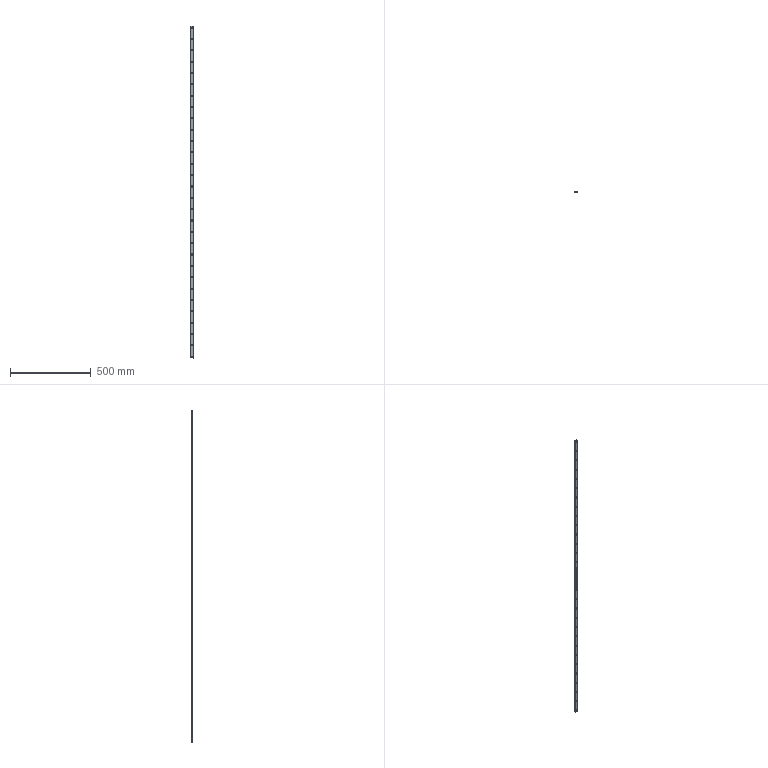Component | SolidWorks | DriveBar-1 | 1 solid | 74 faces | box 18 x 5.2 x 2059.97 mm | volume 125461 mm3 | cylinder 64 | plane 10 | commonest cylinder face diameters 7 x60 1 x4
build123d program:
from build123d import *

# Parameters (mm, degrees)
BOSS_EXTRUDE1_DEPTH     = 2150
SKETCH3_R               = 3.5
CUT_EXTRUDE1_DEPTH      = 53
FILLET1_R               = 0.5
CUT_EXTRUDE2_DEPTH      = 2151.077
CUT_EXTRUDE2_DEPTH_BACK = 2151.077
SKETCH4_W               = 133.386
SKETCH4_H               = 127.729


with BuildPart() as part:
    # Sketch2 → Boss-Extrude1 (new body)
    with BuildSketch(Plane(origin=(0, 0, 0), x_dir=(0, 0, -1), z_dir=(1, 0, 0))):
        Polygon((0, 18), (0, 0), (5.2, 0), (5.2, 2), (3, 2), (3, 16), (5.2, 16), (5.2, 18), align=None)
    extrude(amount=BOSS_EXTRUDE1_DEPTH)

    # Sketch3 → Cut-Extrude1 (cut)
    with BuildSketch(Plane.XY):
        with Locations((10, 9)):
            Circle(SKETCH3_R)
        with Locations((80.4, 9)):
            Circle(SKETCH3_R)
        with Locations((150.8, 9)):
            Circle(SKETCH3_R)
        with Locations((221.2, 9)):
            Circle(SKETCH3_R)
        with Locations((291.6, 9)):
            Circle(SKETCH3_R)
        with Locations((362, 9)):
            Circle(SKETCH3_R)
        with Locations((432.4, 9)):
            Circle(SKETCH3_R)
        with Locations((502.8, 9)):
            Circle(SKETCH3_R)
        with Locations((573.2, 9)):
            Circle(SKETCH3_R)
        with Locations((643.6, 9)):
            Circle(SKETCH3_R)
        with Locations((714, 9)):
            Circle(SKETCH3_R)
        with Locations((784.4, 9)):
            Circle(SKETCH3_R)
        with Locations((854.8, 9)):
            Circle(SKETCH3_R)
        with Locations((925.2, 9)):
            Circle(SKETCH3_R)
        with Locations((995.6, 9)):
            Circle(SKETCH3_R)
        with Locations((1066, 9)):
            Circle(SKETCH3_R)
        with Locations((1136.4, 9)):
            Circle(SKETCH3_R)
        with Locations((1206.8, 9)):
            Circle(SKETCH3_R)
        with Locations((1277.2, 9)):
            Circle(SKETCH3_R)
        with Locations((1347.6, 9)):
            Circle(SKETCH3_R)
        with Locations((1418, 9)):
            Circle(SKETCH3_R)
        with Locations((1488.4, 9)):
            Circle(SKETCH3_R)
        with Locations((1558.8, 9)):
            Circle(SKETCH3_R)
        with Locations((1629.2, 9)):
            Circle(SKETCH3_R)
        with Locations((1699.6, 9)):
            Circle(SKETCH3_R)
        with Locations((1770, 9)):
            Circle(SKETCH3_R)
        with Locations((1840.4, 9)):
            Circle(SKETCH3_R)
        with Locations((1910.8, 9)):
            Circle(SKETCH3_R)
        with Locations((1981.2, 9)):
            Circle(SKETCH3_R)
        with Locations((2051.6, 9)):
            Circle(SKETCH3_R)
        with Locations((2122, 9)):
            Circle(SKETCH3_R)
    extrude(amount=-CUT_EXTRUDE1_DEPTH, mode=Mode.SUBTRACT)

    # Fillet1
    fillet1_edges = [part.edges().sort_by_distance(p)[0] for p in [
        (1075, 18, -5.2),
        (1075, 16, -5.2),
        (1075, 2, -5.2),
        (1075, 0, -5.2),
    ]]
    fillet(fillet1_edges, radius=FILLET1_R)

    # Sketch4 → Cut-Extrude2 (cut, two sides: drawn at the far end of the back side and taken through both)
    with BuildSketch(Plane(origin=(0, 0, -3), x_dir=(-1, 0, 0), z_dir=(0, 0, -1)).offset(-CUT_EXTRUDE2_DEPTH_BACK)):
        with Locations((-2126.667, 12.853)):
            Rectangle(SKETCH4_W, SKETCH4_H)
    extrude(amount=CUT_EXTRUDE2_DEPTH + CUT_EXTRUDE2_DEPTH_BACK, mode=Mode.SUBTRACT)


solid = part.part

# Placed as in the assembly
solid = solid.moved(Location((55.241, 20.247, 1782.648), (90, 0, -90)))